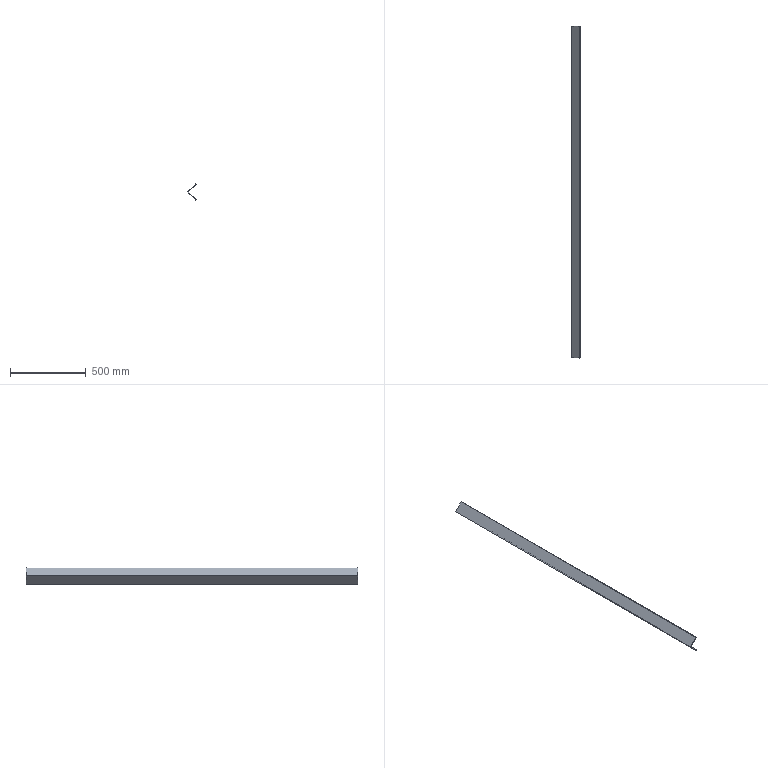Component | NX | CANTONEIRA | 1 solid | 12 faces | box 56.59 x 2190 x 106.11 mm | volume 1606510 mm3 | plane 8 | cylinder 4 | commonest cylinder face diameters 4 x4
STEP:
#1=CARTESIAN_POINT('',(0.,0.,0.));
#2=DIRECTION('',(0.,0.,1.));
#3=DIRECTION('',(1.,0.,0.));
#4=AXIS2_PLACEMENT_3D('',#1,#2,#3);
#5=CARTESIAN_POINT('',(-19.121,755.233,574.48));
#6=VERTEX_POINT('',#5);
#7=CARTESIAN_POINT('',(-71.589,755.233,626.947));
#8=VERTEX_POINT('',#7);
#9=CARTESIAN_POINT('',(-17.707,755.233,573.065));
#10=DIRECTION('',(-0.7071,0.,0.7071));
#11=VECTOR('',#10,1.);
#12=LINE('',#9,#11);
#13=CARTESIAN_POINT('',(-17.707,755.233,573.065));
#14=DIRECTION('',(0.7071,0.,0.7071));
#15=DIRECTION('',(-0.7071,0.,0.7071));
#16=AXIS2_PLACEMENT_3D('',#13,#14,#15);
#17=PLANE('',#16);
#18=CARTESIAN_POINT('',(0.,0.));
#19=DIRECTION('',(1.,0.));
#20=VECTOR('',#19,1.);
#21=LINE('',#18,#20);
#22=(GEOMETRIC_REPRESENTATION_CONTEXT(2)PARAMETRIC_REPRESENTATION_CONTEXT()REPRESENTATION_CONTEXT('',''));
#23=DEFINITIONAL_REPRESENTATION('',(#21),#22);
#24=PCURVE('',#17,#23);
#25=CARTESIAN_POINT('',(-71.589,755.233,626.947));
#26=DIRECTION('',(0.,1.,0.));
#27=DIRECTION('',(-0.7071,0.,0.7071));
#28=AXIS2_PLACEMENT_3D('',#25,#26,#27);
#29=PLANE('',#28);
#30=CARTESIAN_POINT('',(-76.2,0.));
#31=DIRECTION('',(1.,0.));
#32=VECTOR('',#31,1.);
#33=LINE('',#30,#32);
#34=(GEOMETRIC_REPRESENTATION_CONTEXT(2)PARAMETRIC_REPRESENTATION_CONTEXT()REPRESENTATION_CONTEXT('',''));
#35=DEFINITIONAL_REPRESENTATION('',(#33),#34);
#36=PCURVE('',#29,#35);
#37=SURFACE_CURVE('',#12,(#24,#36),.PCURVE_S1.);
#38=EDGE_CURVE('',#6,#8,#37,.T.);
#39=ORIENTED_EDGE('',*,*,#38,.F.);
#40=CARTESIAN_POINT('',(-19.121,-1434.767,574.48));
#41=VERTEX_POINT('',#40);
#42=CARTESIAN_POINT('',(-19.121,755.233,574.48));
#43=DIRECTION('',(0.,-1.,0.));
#44=VECTOR('',#43,1.);
#45=LINE('',#42,#44);
#46=CARTESIAN_POINT('',(2.,0.));
#47=DIRECTION('',(0.,1.));
#48=VECTOR('',#47,1.);
#49=LINE('',#46,#48);
#50=(GEOMETRIC_REPRESENTATION_CONTEXT(2)PARAMETRIC_REPRESENTATION_CONTEXT()REPRESENTATION_CONTEXT('',''));
#51=DEFINITIONAL_REPRESENTATION('',(#49),#50);
#52=PCURVE('',#17,#51);
#53=CARTESIAN_POINT('',(-17.707,755.233,575.894));
#54=DIRECTION('',(0.,-1.,0.));
#55=DIRECTION('',(0.7071,0.,-0.7071));
#56=AXIS2_PLACEMENT_3D('',#53,#54,#55);
#57=CYLINDRICAL_SURFACE('',#56,2.);
#58=CARTESIAN_POINT('',(4.712,0.));
#59=DIRECTION('',(0.,1.));
#60=VECTOR('',#59,1.);
#61=LINE('',#58,#60);
#62=(GEOMETRIC_REPRESENTATION_CONTEXT(2)PARAMETRIC_REPRESENTATION_CONTEXT()REPRESENTATION_CONTEXT('',''));
#63=DEFINITIONAL_REPRESENTATION('',(#61),#62);
#64=PCURVE('',#57,#63);
#65=SURFACE_CURVE('',#45,(#52,#64),.PCURVE_S1.);
#66=EDGE_CURVE('',#6,#41,#65,.T.);
#67=ORIENTED_EDGE('',*,*,#66,.T.);
#68=CARTESIAN_POINT('',(-71.589,-1434.767,626.947));
#69=VERTEX_POINT('',#68);
#70=CARTESIAN_POINT('',(-17.707,-1434.767,573.065));
#71=DIRECTION('',(-0.7071,0.,0.7071));
#72=VECTOR('',#71,1.);
#73=LINE('',#70,#72);
#74=CARTESIAN_POINT('',(0.,2190.));
#75=DIRECTION('',(1.,0.));
#76=VECTOR('',#75,1.);
#77=LINE('',#74,#76);
#78=(GEOMETRIC_REPRESENTATION_CONTEXT(2)PARAMETRIC_REPRESENTATION_CONTEXT()REPRESENTATION_CONTEXT('',''));
#79=DEFINITIONAL_REPRESENTATION('',(#77),#78);
#80=PCURVE('',#17,#79);
#81=CARTESIAN_POINT('',(-71.589,-1434.767,626.947));
#82=DIRECTION('',(0.,1.,0.));
#83=DIRECTION('',(-0.7071,0.,0.7071));
#84=AXIS2_PLACEMENT_3D('',#81,#82,#83);
#85=PLANE('',#84);
#86=CARTESIAN_POINT('',(-76.2,0.));
#87=DIRECTION('',(1.,0.));
#88=VECTOR('',#87,1.);
#89=LINE('',#86,#88);
#90=(GEOMETRIC_REPRESENTATION_CONTEXT(2)PARAMETRIC_REPRESENTATION_CONTEXT()REPRESENTATION_CONTEXT('',''));
#91=DEFINITIONAL_REPRESENTATION('',(#89),#90);
#92=PCURVE('',#85,#91);
#93=SURFACE_CURVE('',#73,(#80,#92),.PCURVE_S1.);
#94=EDGE_CURVE('',#41,#69,#93,.T.);
#95=ORIENTED_EDGE('',*,*,#94,.T.);
#96=CARTESIAN_POINT('',(-71.589,755.233,626.947));
#97=DIRECTION('',(0.,-1.,0.));
#98=VECTOR('',#97,1.);
#99=LINE('',#96,#98);
#100=CARTESIAN_POINT('',(76.2,0.));
#101=DIRECTION('',(0.,1.));
#102=VECTOR('',#101,1.);
#103=LINE('',#100,#102);
#104=(GEOMETRIC_REPRESENTATION_CONTEXT(2)PARAMETRIC_REPRESENTATION_CONTEXT()REPRESENTATION_CONTEXT('',''));
#105=DEFINITIONAL_REPRESENTATION('',(#103),#104);
#106=PCURVE('',#17,#105);
#107=CARTESIAN_POINT('',(-71.589,755.233,626.947));
#108=DIRECTION('',(0.7071,0.,-0.7071));
#109=DIRECTION('',(0.7071,0.,0.7071));
#110=AXIS2_PLACEMENT_3D('',#107,#108,#109);
#111=PLANE('',#110);
#112=CARTESIAN_POINT('',(0.,0.));
#113=DIRECTION('',(0.,1.));
#114=VECTOR('',#113,1.);
#115=LINE('',#112,#114);
#116=(GEOMETRIC_REPRESENTATION_CONTEXT(2)PARAMETRIC_REPRESENTATION_CONTEXT()REPRESENTATION_CONTEXT('',''));
#117=DEFINITIONAL_REPRESENTATION('',(#115),#116);
#118=PCURVE('',#111,#117);
#119=SURFACE_CURVE('',#99,(#106,#118),.PCURVE_S1.);
#120=EDGE_CURVE('',#8,#69,#119,.T.);
#121=ORIENTED_EDGE('',*,*,#120,.F.);
#122=EDGE_LOOP('',(#39,#67,#95,#121));
#123=FACE_BOUND('',#122,.T.);
#124=ADVANCED_FACE('',(#123),#17,.F.);
#125=CARTESIAN_POINT('',(-19.121,-1434.767,679.414));
#126=VERTEX_POINT('',#125);
#127=CARTESIAN_POINT('',(-71.589,-1434.767,626.947));
#128=DIRECTION('',(0.7071,0.,0.7071));
#129=VECTOR('',#128,1.);
#130=LINE('',#127,#129);
#131=CARTESIAN_POINT('',(0.,2190.));
#132=DIRECTION('',(1.,0.));
#133=VECTOR('',#132,1.);
#134=LINE('',#131,#133);
#135=(GEOMETRIC_REPRESENTATION_CONTEXT(2)PARAMETRIC_REPRESENTATION_CONTEXT()REPRESENTATION_CONTEXT('',''));
#136=DEFINITIONAL_REPRESENTATION('',(#134),#135);
#137=PCURVE('',#111,#136);
#138=CARTESIAN_POINT('',(0.,0.));
#139=DIRECTION('',(0.,1.));
#140=VECTOR('',#139,1.);
#141=LINE('',#138,#140);
#142=(GEOMETRIC_REPRESENTATION_CONTEXT(2)PARAMETRIC_REPRESENTATION_CONTEXT()REPRESENTATION_CONTEXT('',''));
#143=DEFINITIONAL_REPRESENTATION('',(#141),#142);
#144=PCURVE('',#85,#143);
#145=SURFACE_CURVE('',#130,(#137,#144),.PCURVE_S1.);
#146=EDGE_CURVE('',#69,#126,#145,.T.);
#147=ORIENTED_EDGE('',*,*,#146,.T.);
#148=CARTESIAN_POINT('',(-19.121,755.233,679.414));
#149=VERTEX_POINT('',#148);
#150=CARTESIAN_POINT('',(-19.121,755.233,679.414));
#151=DIRECTION('',(0.,1.,0.));
#152=VECTOR('',#151,1.);
#153=LINE('',#150,#152);
#154=CARTESIAN_POINT('',(74.2,0.));
#155=DIRECTION('',(0.,-1.));
#156=VECTOR('',#155,1.);
#157=LINE('',#154,#156);
#158=(GEOMETRIC_REPRESENTATION_CONTEXT(2)PARAMETRIC_REPRESENTATION_CONTEXT()REPRESENTATION_CONTEXT('',''));
#159=DEFINITIONAL_REPRESENTATION('',(#157),#158);
#160=PCURVE('',#111,#159);
#161=CARTESIAN_POINT('',(-17.707,755.233,678.));
#162=DIRECTION('',(0.,-1.,0.));
#163=DIRECTION('',(0.7071,0.,-0.7071));
#164=AXIS2_PLACEMENT_3D('',#161,#162,#163);
#165=CYLINDRICAL_SURFACE('',#164,2.);
#166=CARTESIAN_POINT('',(3.142,0.));
#167=DIRECTION('',(0.,-1.));
#168=VECTOR('',#167,1.);
#169=LINE('',#166,#168);
#170=(GEOMETRIC_REPRESENTATION_CONTEXT(2)PARAMETRIC_REPRESENTATION_CONTEXT()REPRESENTATION_CONTEXT('',''));
#171=DEFINITIONAL_REPRESENTATION('',(#169),#170);
#172=PCURVE('',#165,#171);
#173=SURFACE_CURVE('',#153,(#160,#172),.PCURVE_S1.);
#174=EDGE_CURVE('',#126,#149,#173,.T.);
#175=ORIENTED_EDGE('',*,*,#174,.T.);
#176=CARTESIAN_POINT('',(-71.589,755.233,626.947));
#177=DIRECTION('',(0.7071,0.,0.7071));
#178=VECTOR('',#177,1.);
#179=LINE('',#176,#178);
#180=CARTESIAN_POINT('',(0.,0.));
#181=DIRECTION('',(1.,0.));
#182=VECTOR('',#181,1.);
#183=LINE('',#180,#182);
#184=(GEOMETRIC_REPRESENTATION_CONTEXT(2)PARAMETRIC_REPRESENTATION_CONTEXT()REPRESENTATION_CONTEXT('',''));
#185=DEFINITIONAL_REPRESENTATION('',(#183),#184);
#186=PCURVE('',#111,#185);
#187=CARTESIAN_POINT('',(0.,0.));
#188=DIRECTION('',(0.,1.));
#189=VECTOR('',#188,1.);
#190=LINE('',#187,#189);
#191=(GEOMETRIC_REPRESENTATION_CONTEXT(2)PARAMETRIC_REPRESENTATION_CONTEXT()REPRESENTATION_CONTEXT('',''));
#192=DEFINITIONAL_REPRESENTATION('',(#190),#191);
#193=PCURVE('',#29,#192);
#194=SURFACE_CURVE('',#179,(#186,#193),.PCURVE_S1.);
#195=EDGE_CURVE('',#8,#149,#194,.T.);
#196=ORIENTED_EDGE('',*,*,#195,.F.);
#197=ORIENTED_EDGE('',*,*,#120,.T.);
#198=EDGE_LOOP('',(#147,#175,#196,#197));
#199=FACE_BOUND('',#198,.T.);
#200=ADVANCED_FACE('',(#199),#111,.F.);
#201=CARTESIAN_POINT('',(-16.293,755.233,679.414));
#202=VERTEX_POINT('',#201);
#203=CARTESIAN_POINT('',(-15.586,755.233,678.707));
#204=VERTEX_POINT('',#203);
#205=CARTESIAN_POINT('',(-17.707,755.233,680.828));
#206=DIRECTION('',(0.7071,0.,-0.7071));
#207=VECTOR('',#206,1.);
#208=LINE('',#205,#207);
#209=CARTESIAN_POINT('',(-17.707,755.233,680.828));
#210=DIRECTION('',(-0.7071,0.,-0.7071));
#211=DIRECTION('',(0.7071,0.,-0.7071));
#212=AXIS2_PLACEMENT_3D('',#209,#210,#211);
#213=PLANE('',#212);
#214=CARTESIAN_POINT('',(0.,0.));
#215=DIRECTION('',(1.,0.));
#216=VECTOR('',#215,1.);
#217=LINE('',#214,#216);
#218=(GEOMETRIC_REPRESENTATION_CONTEXT(2)PARAMETRIC_REPRESENTATION_CONTEXT()REPRESENTATION_CONTEXT('',''));
#219=DEFINITIONAL_REPRESENTATION('',(#217),#218);
#220=PCURVE('',#213,#219);
#221=CARTESIAN_POINT('',(-0.,76.2));
#222=DIRECTION('',(-1.,0.));
#223=VECTOR('',#222,1.);
#224=LINE('',#221,#223);
#225=(GEOMETRIC_REPRESENTATION_CONTEXT(2)PARAMETRIC_REPRESENTATION_CONTEXT()REPRESENTATION_CONTEXT('',''));
#226=DEFINITIONAL_REPRESENTATION('',(#224),#225);
#227=PCURVE('',#29,#226);
#228=SURFACE_CURVE('',#208,(#220,#227),.PCURVE_S1.);
#229=EDGE_CURVE('',#202,#204,#228,.T.);
#230=ORIENTED_EDGE('',*,*,#229,.F.);
#231=CARTESIAN_POINT('',(-16.293,-1434.767,679.414));
#232=VERTEX_POINT('',#231);
#233=CARTESIAN_POINT('',(-16.293,755.233,679.414));
#234=DIRECTION('',(0.,-1.,0.));
#235=VECTOR('',#234,1.);
#236=LINE('',#233,#235);
#237=CARTESIAN_POINT('',(2.,0.));
#238=DIRECTION('',(0.,1.));
#239=VECTOR('',#238,1.);
#240=LINE('',#237,#239);
#241=(GEOMETRIC_REPRESENTATION_CONTEXT(2)PARAMETRIC_REPRESENTATION_CONTEXT()REPRESENTATION_CONTEXT('',''));
#242=DEFINITIONAL_REPRESENTATION('',(#240),#241);
#243=PCURVE('',#213,#242);
#244=CARTESIAN_POINT('',(1.571,0.));
#245=DIRECTION('',(0.,1.));
#246=VECTOR('',#245,1.);
#247=LINE('',#244,#246);
#248=(GEOMETRIC_REPRESENTATION_CONTEXT(2)PARAMETRIC_REPRESENTATION_CONTEXT()REPRESENTATION_CONTEXT('',''));
#249=DEFINITIONAL_REPRESENTATION('',(#247),#248);
#250=PCURVE('',#165,#249);
#251=SURFACE_CURVE('',#236,(#243,#250),.PCURVE_S1.);
#252=EDGE_CURVE('',#202,#232,#251,.T.);
#253=ORIENTED_EDGE('',*,*,#252,.T.);
#254=CARTESIAN_POINT('',(-15.586,-1434.767,678.707));
#255=VERTEX_POINT('',#254);
#256=CARTESIAN_POINT('',(-17.707,-1434.767,680.828));
#257=DIRECTION('',(0.7071,0.,-0.7071));
#258=VECTOR('',#257,1.);
#259=LINE('',#256,#258);
#260=CARTESIAN_POINT('',(0.,2190.));
#261=DIRECTION('',(1.,0.));
#262=VECTOR('',#261,1.);
#263=LINE('',#260,#262);
#264=(GEOMETRIC_REPRESENTATION_CONTEXT(2)PARAMETRIC_REPRESENTATION_CONTEXT()REPRESENTATION_CONTEXT('',''));
#265=DEFINITIONAL_REPRESENTATION('',(#263),#264);
#266=PCURVE('',#213,#265);
#267=CARTESIAN_POINT('',(-0.,76.2));
#268=DIRECTION('',(-1.,0.));
#269=VECTOR('',#268,1.);
#270=LINE('',#267,#269);
#271=(GEOMETRIC_REPRESENTATION_CONTEXT(2)PARAMETRIC_REPRESENTATION_CONTEXT()REPRESENTATION_CONTEXT('',''));
#272=DEFINITIONAL_REPRESENTATION('',(#270),#271);
#273=PCURVE('',#85,#272);
#274=SURFACE_CURVE('',#259,(#266,#273),.PCURVE_S1.);
#275=EDGE_CURVE('',#232,#255,#274,.T.);
#276=ORIENTED_EDGE('',*,*,#275,.T.);
#277=CARTESIAN_POINT('',(-15.586,755.233,678.707));
#278=DIRECTION('',(0.,1.,0.));
#279=VECTOR('',#278,1.);
#280=LINE('',#277,#279);
#281=CARTESIAN_POINT('',(3.,0.));
#282=DIRECTION('',(0.,-1.));
#283=VECTOR('',#282,1.);
#284=LINE('',#281,#283);
#285=(GEOMETRIC_REPRESENTATION_CONTEXT(2)PARAMETRIC_REPRESENTATION_CONTEXT()REPRESENTATION_CONTEXT('',''));
#286=DEFINITIONAL_REPRESENTATION('',(#284),#285);
#287=PCURVE('',#213,#286);
#288=CARTESIAN_POINT('',(-17.,755.233,677.293));
#289=DIRECTION('',(0.,-1.,0.));
#290=DIRECTION('',(0.7071,0.,-0.7071));
#291=AXIS2_PLACEMENT_3D('',#288,#289,#290);
#292=CYLINDRICAL_SURFACE('',#291,2.);
#293=CARTESIAN_POINT('',(1.571,0.));
#294=DIRECTION('',(0.,-1.));
#295=VECTOR('',#294,1.);
#296=LINE('',#293,#295);
#297=(GEOMETRIC_REPRESENTATION_CONTEXT(2)PARAMETRIC_REPRESENTATION_CONTEXT()REPRESENTATION_CONTEXT('',''));
#298=DEFINITIONAL_REPRESENTATION('',(#296),#297);
#299=PCURVE('',#292,#298);
#300=SURFACE_CURVE('',#280,(#287,#299),.PCURVE_S1.);
#301=EDGE_CURVE('',#255,#204,#300,.T.);
#302=ORIENTED_EDGE('',*,*,#301,.T.);
#303=EDGE_LOOP('',(#230,#253,#276,#302));
#304=FACE_BOUND('',#303,.T.);
#305=ADVANCED_FACE('',(#304),#213,.F.);
#306=CARTESIAN_POINT('',(-15.586,755.233,675.879));
#307=VERTEX_POINT('',#306);
#308=CARTESIAN_POINT('',(-64.518,755.233,626.947));
#309=VERTEX_POINT('',#308);
#310=CARTESIAN_POINT('',(-14.172,755.233,677.293));
#311=DIRECTION('',(-0.7071,0.,-0.7071));
#312=VECTOR('',#311,1.);
#313=LINE('',#310,#312);
#314=CARTESIAN_POINT('',(-14.172,755.233,677.293));
#315=DIRECTION('',(-0.7071,0.,0.7071));
#316=DIRECTION('',(-0.7071,0.,-0.7071));
#317=AXIS2_PLACEMENT_3D('',#314,#315,#316);
#318=PLANE('',#317);
#319=CARTESIAN_POINT('',(0.,0.));
#320=DIRECTION('',(1.,0.));
#321=VECTOR('',#320,1.);
#322=LINE('',#319,#321);
#323=(GEOMETRIC_REPRESENTATION_CONTEXT(2)PARAMETRIC_REPRESENTATION_CONTEXT()REPRESENTATION_CONTEXT('',''));
#324=DEFINITIONAL_REPRESENTATION('',(#322),#323);
#325=PCURVE('',#318,#324);
#326=CARTESIAN_POINT('',(-5.,76.2));
#327=DIRECTION('',(0.,-1.));
#328=VECTOR('',#327,1.);
#329=LINE('',#326,#328);
#330=(GEOMETRIC_REPRESENTATION_CONTEXT(2)PARAMETRIC_REPRESENTATION_CONTEXT()REPRESENTATION_CONTEXT('',''));
#331=DEFINITIONAL_REPRESENTATION('',(#329),#330);
#332=PCURVE('',#29,#331);
#333=SURFACE_CURVE('',#313,(#325,#332),.PCURVE_S1.);
#334=EDGE_CURVE('',#307,#309,#333,.T.);
#335=ORIENTED_EDGE('',*,*,#334,.F.);
#336=CARTESIAN_POINT('',(-15.586,-1434.767,675.879));
#337=VERTEX_POINT('',#336);
#338=CARTESIAN_POINT('',(-15.586,755.233,675.879));
#339=DIRECTION('',(0.,-1.,0.));
#340=VECTOR('',#339,1.);
#341=LINE('',#338,#340);
#342=CARTESIAN_POINT('',(2.,0.));
#343=DIRECTION('',(0.,1.));
#344=VECTOR('',#343,1.);
#345=LINE('',#342,#344);
#346=(GEOMETRIC_REPRESENTATION_CONTEXT(2)PARAMETRIC_REPRESENTATION_CONTEXT()REPRESENTATION_CONTEXT('',''));
#347=DEFINITIONAL_REPRESENTATION('',(#345),#346);
#348=PCURVE('',#318,#347);
#349=CARTESIAN_POINT('',(0.,0.));
#350=DIRECTION('',(0.,1.));
#351=VECTOR('',#350,1.);
#352=LINE('',#349,#351);
#353=(GEOMETRIC_REPRESENTATION_CONTEXT(2)PARAMETRIC_REPRESENTATION_CONTEXT()REPRESENTATION_CONTEXT('',''));
#354=DEFINITIONAL_REPRESENTATION('',(#352),#353);
#355=PCURVE('',#292,#354);
#356=SURFACE_CURVE('',#341,(#348,#355),.PCURVE_S1.);
#357=EDGE_CURVE('',#307,#337,#356,.T.);
#358=ORIENTED_EDGE('',*,*,#357,.T.);
#359=CARTESIAN_POINT('',(-64.518,-1434.767,626.947));
#360=VERTEX_POINT('',#359);
#361=CARTESIAN_POINT('',(-14.172,-1434.767,677.293));
#362=DIRECTION('',(-0.7071,0.,-0.7071));
#363=VECTOR('',#362,1.);
#364=LINE('',#361,#363);
#365=CARTESIAN_POINT('',(0.,2190.));
#366=DIRECTION('',(1.,0.));
#367=VECTOR('',#366,1.);
#368=LINE('',#365,#367);
#369=(GEOMETRIC_REPRESENTATION_CONTEXT(2)PARAMETRIC_REPRESENTATION_CONTEXT()REPRESENTATION_CONTEXT('',''));
#370=DEFINITIONAL_REPRESENTATION('',(#368),#369);
#371=PCURVE('',#318,#370);
#372=CARTESIAN_POINT('',(-5.,76.2));
#373=DIRECTION('',(0.,-1.));
#374=VECTOR('',#373,1.);
#375=LINE('',#372,#374);
#376=(GEOMETRIC_REPRESENTATION_CONTEXT(2)PARAMETRIC_REPRESENTATION_CONTEXT()REPRESENTATION_CONTEXT('',''));
#377=DEFINITIONAL_REPRESENTATION('',(#375),#376);
#378=PCURVE('',#85,#377);
#379=SURFACE_CURVE('',#364,(#371,#378),.PCURVE_S1.);
#380=EDGE_CURVE('',#337,#360,#379,.T.);
#381=ORIENTED_EDGE('',*,*,#380,.T.);
#382=CARTESIAN_POINT('',(-64.518,755.233,626.947));
#383=DIRECTION('',(0.,-1.,0.));
#384=VECTOR('',#383,1.);
#385=LINE('',#382,#384);
#386=CARTESIAN_POINT('',(71.2,0.));
#387=DIRECTION('',(0.,1.));
#388=VECTOR('',#387,1.);
#389=LINE('',#386,#388);
#390=(GEOMETRIC_REPRESENTATION_CONTEXT(2)PARAMETRIC_REPRESENTATION_CONTEXT()REPRESENTATION_CONTEXT('',''));
#391=DEFINITIONAL_REPRESENTATION('',(#389),#390);
#392=PCURVE('',#318,#391);
#393=CARTESIAN_POINT('',(-64.518,755.233,626.947));
#394=DIRECTION('',(-0.7071,0.,-0.7071));
#395=DIRECTION('',(0.7071,0.,-0.7071));
#396=AXIS2_PLACEMENT_3D('',#393,#394,#395);
#397=PLANE('',#396);
#398=CARTESIAN_POINT('',(0.,0.));
#399=DIRECTION('',(0.,1.));
#400=VECTOR('',#399,1.);
#401=LINE('',#398,#400);
#402=(GEOMETRIC_REPRESENTATION_CONTEXT(2)PARAMETRIC_REPRESENTATION_CONTEXT()REPRESENTATION_CONTEXT('',''));
#403=DEFINITIONAL_REPRESENTATION('',(#401),#402);
#404=PCURVE('',#397,#403);
#405=SURFACE_CURVE('',#385,(#392,#404),.PCURVE_S1.);
#406=EDGE_CURVE('',#309,#360,#405,.T.);
#407=ORIENTED_EDGE('',*,*,#406,.F.);
#408=EDGE_LOOP('',(#335,#358,#381,#407));
#409=FACE_BOUND('',#408,.T.);
#410=ADVANCED_FACE('',(#409),#318,.F.);
#411=CARTESIAN_POINT('',(-15.586,-1434.767,578.015));
#412=VERTEX_POINT('',#411);
#413=CARTESIAN_POINT('',(-64.518,-1434.767,626.947));
#414=DIRECTION('',(0.7071,0.,-0.7071));
#415=VECTOR('',#414,1.);
#416=LINE('',#413,#415);
#417=CARTESIAN_POINT('',(0.,2190.));
#418=DIRECTION('',(1.,0.));
#419=VECTOR('',#418,1.);
#420=LINE('',#417,#419);
#421=(GEOMETRIC_REPRESENTATION_CONTEXT(2)PARAMETRIC_REPRESENTATION_CONTEXT()REPRESENTATION_CONTEXT('',''));
#422=DEFINITIONAL_REPRESENTATION('',(#420),#421);
#423=PCURVE('',#397,#422);
#424=CARTESIAN_POINT('',(-5.,5.));
#425=DIRECTION('',(-1.,0.));
#426=VECTOR('',#425,1.);
#427=LINE('',#424,#426);
#428=(GEOMETRIC_REPRESENTATION_CONTEXT(2)PARAMETRIC_REPRESENTATION_CONTEXT()REPRESENTATION_CONTEXT('',''));
#429=DEFINITIONAL_REPRESENTATION('',(#427),#428);
#430=PCURVE('',#85,#429);
#431=SURFACE_CURVE('',#416,(#423,#430),.PCURVE_S1.);
#432=EDGE_CURVE('',#360,#412,#431,.T.);
#433=ORIENTED_EDGE('',*,*,#432,.T.);
#434=CARTESIAN_POINT('',(-15.586,755.233,578.015));
#435=VERTEX_POINT('',#434);
#436=CARTESIAN_POINT('',(-15.586,755.233,578.015));
#437=DIRECTION('',(0.,1.,0.));
#438=VECTOR('',#437,1.);
#439=LINE('',#436,#438);
#440=CARTESIAN_POINT('',(69.2,0.));
#441=DIRECTION('',(0.,-1.));
#442=VECTOR('',#441,1.);
#443=LINE('',#440,#442);
#444=(GEOMETRIC_REPRESENTATION_CONTEXT(2)PARAMETRIC_REPRESENTATION_CONTEXT()REPRESENTATION_CONTEXT('',''));
#445=DEFINITIONAL_REPRESENTATION('',(#443),#444);
#446=PCURVE('',#397,#445);
#447=CARTESIAN_POINT('',(-17.,755.233,576.601));
#448=DIRECTION('',(0.,-1.,0.));
#449=DIRECTION('',(0.7071,0.,-0.7071));
#450=AXIS2_PLACEMENT_3D('',#447,#448,#449);
#451=CYLINDRICAL_SURFACE('',#450,2.);
#452=CARTESIAN_POINT('',(1.571,0.));
#453=DIRECTION('',(0.,-1.));
#454=VECTOR('',#453,1.);
#455=LINE('',#452,#454);
#456=(GEOMETRIC_REPRESENTATION_CONTEXT(2)PARAMETRIC_REPRESENTATION_CONTEXT()REPRESENTATION_CONTEXT('',''));
#457=DEFINITIONAL_REPRESENTATION('',(#455),#456);
#458=PCURVE('',#451,#457);
#459=SURFACE_CURVE('',#439,(#446,#458),.PCURVE_S1.);
#460=EDGE_CURVE('',#412,#435,#459,.T.);
#461=ORIENTED_EDGE('',*,*,#460,.T.);
#462=CARTESIAN_POINT('',(-64.518,755.233,626.947));
#463=DIRECTION('',(0.7071,0.,-0.7071));
#464=VECTOR('',#463,1.);
#465=LINE('',#462,#464);
#466=CARTESIAN_POINT('',(0.,0.));
#467=DIRECTION('',(1.,0.));
#468=VECTOR('',#467,1.);
#469=LINE('',#466,#468);
#470=(GEOMETRIC_REPRESENTATION_CONTEXT(2)PARAMETRIC_REPRESENTATION_CONTEXT()REPRESENTATION_CONTEXT('',''));
#471=DEFINITIONAL_REPRESENTATION('',(#469),#470);
#472=PCURVE('',#397,#471);
#473=CARTESIAN_POINT('',(-5.,5.));
#474=DIRECTION('',(-1.,0.));
#475=VECTOR('',#474,1.);
#476=LINE('',#473,#475);
#477=(GEOMETRIC_REPRESENTATION_CONTEXT(2)PARAMETRIC_REPRESENTATION_CONTEXT()REPRESENTATION_CONTEXT('',''));
#478=DEFINITIONAL_REPRESENTATION('',(#476),#477);
#479=PCURVE('',#29,#478);
#480=SURFACE_CURVE('',#465,(#472,#479),.PCURVE_S1.);
#481=EDGE_CURVE('',#309,#435,#480,.T.);
#482=ORIENTED_EDGE('',*,*,#481,.F.);
#483=ORIENTED_EDGE('',*,*,#406,.T.);
#484=EDGE_LOOP('',(#433,#461,#482,#483));
#485=FACE_BOUND('',#484,.T.);
#486=ADVANCED_FACE('',(#485),#397,.F.);
#487=CARTESIAN_POINT('',(-15.586,755.233,575.187));
#488=VERTEX_POINT('',#487);
#489=CARTESIAN_POINT('',(-16.293,755.233,574.48));
#490=VERTEX_POINT('',#489);
#491=CARTESIAN_POINT('',(-14.172,755.233,576.601));
#492=DIRECTION('',(-0.7071,0.,-0.7071));
#493=VECTOR('',#492,1.);
#494=LINE('',#491,#493);
#495=CARTESIAN_POINT('',(-14.172,755.233,576.601));
#496=DIRECTION('',(-0.7071,0.,0.7071));
#497=DIRECTION('',(-0.7071,0.,-0.7071));
#498=AXIS2_PLACEMENT_3D('',#495,#496,#497);
#499=PLANE('',#498);
#500=CARTESIAN_POINT('',(0.,0.));
#501=DIRECTION('',(1.,0.));
#502=VECTOR('',#501,1.);
#503=LINE('',#500,#502);
#504=(GEOMETRIC_REPRESENTATION_CONTEXT(2)PARAMETRIC_REPRESENTATION_CONTEXT()REPRESENTATION_CONTEXT('',''));
#505=DEFINITIONAL_REPRESENTATION('',(#503),#504);
#506=PCURVE('',#499,#505);
#507=CARTESIAN_POINT('',(-76.2,5.));
#508=DIRECTION('',(0.,-1.));
#509=VECTOR('',#508,1.);
#510=LINE('',#507,#509);
#511=(GEOMETRIC_REPRESENTATION_CONTEXT(2)PARAMETRIC_REPRESENTATION_CONTEXT()REPRESENTATION_CONTEXT('',''));
#512=DEFINITIONAL_REPRESENTATION('',(#510),#511);
#513=PCURVE('',#29,#512);
#514=SURFACE_CURVE('',#494,(#506,#513),.PCURVE_S1.);
#515=EDGE_CURVE('',#488,#490,#514,.T.);
#516=ORIENTED_EDGE('',*,*,#515,.F.);
#517=CARTESIAN_POINT('',(-15.586,-1434.767,575.187));
#518=VERTEX_POINT('',#517);
#519=CARTESIAN_POINT('',(-15.586,755.233,575.187));
#520=DIRECTION('',(0.,-1.,0.));
#521=VECTOR('',#520,1.);
#522=LINE('',#519,#521);
#523=CARTESIAN_POINT('',(2.,0.));
#524=DIRECTION('',(0.,1.));
#525=VECTOR('',#524,1.);
#526=LINE('',#523,#525);
#527=(GEOMETRIC_REPRESENTATION_CONTEXT(2)PARAMETRIC_REPRESENTATION_CONTEXT()REPRESENTATION_CONTEXT('',''));
#528=DEFINITIONAL_REPRESENTATION('',(#526),#527);
#529=PCURVE('',#499,#528);
#530=CARTESIAN_POINT('',(0.,0.));
#531=DIRECTION('',(0.,1.));
#532=VECTOR('',#531,1.);
#533=LINE('',#530,#532);
#534=(GEOMETRIC_REPRESENTATION_CONTEXT(2)PARAMETRIC_REPRESENTATION_CONTEXT()REPRESENTATION_CONTEXT('',''));
#535=DEFINITIONAL_REPRESENTATION('',(#533),#534);
#536=PCURVE('',#451,#535);
#537=SURFACE_CURVE('',#522,(#529,#536),.PCURVE_S1.);
#538=EDGE_CURVE('',#488,#518,#537,.T.);
#539=ORIENTED_EDGE('',*,*,#538,.T.);
#540=CARTESIAN_POINT('',(-16.293,-1434.767,574.48));
#541=VERTEX_POINT('',#540);
#542=CARTESIAN_POINT('',(-14.172,-1434.767,576.601));
#543=DIRECTION('',(-0.7071,0.,-0.7071));
#544=VECTOR('',#543,1.);
#545=LINE('',#542,#544);
#546=CARTESIAN_POINT('',(0.,2190.));
#547=DIRECTION('',(1.,0.));
#548=VECTOR('',#547,1.);
#549=LINE('',#546,#548);
#550=(GEOMETRIC_REPRESENTATION_CONTEXT(2)PARAMETRIC_REPRESENTATION_CONTEXT()REPRESENTATION_CONTEXT('',''));
#551=DEFINITIONAL_REPRESENTATION('',(#549),#550);
#552=PCURVE('',#499,#551);
#553=CARTESIAN_POINT('',(-76.2,5.));
#554=DIRECTION('',(0.,-1.));
#555=VECTOR('',#554,1.);
#556=LINE('',#553,#555);
#557=(GEOMETRIC_REPRESENTATION_CONTEXT(2)PARAMETRIC_REPRESENTATION_CONTEXT()REPRESENTATION_CONTEXT('',''));
#558=DEFINITIONAL_REPRESENTATION('',(#556),#557);
#559=PCURVE('',#85,#558);
#560=SURFACE_CURVE('',#545,(#552,#559),.PCURVE_S1.);
#561=EDGE_CURVE('',#518,#541,#560,.T.);
#562=ORIENTED_EDGE('',*,*,#561,.T.);
#563=CARTESIAN_POINT('',(-16.293,755.233,574.48));
#564=DIRECTION('',(0.,1.,0.));
#565=VECTOR('',#564,1.);
#566=LINE('',#563,#565);
#567=CARTESIAN_POINT('',(3.,0.));
#568=DIRECTION('',(0.,-1.));
#569=VECTOR('',#568,1.);
#570=LINE('',#567,#569);
#571=(GEOMETRIC_REPRESENTATION_CONTEXT(2)PARAMETRIC_REPRESENTATION_CONTEXT()REPRESENTATION_CONTEXT('',''));
#572=DEFINITIONAL_REPRESENTATION('',(#570),#571);
#573=PCURVE('',#499,#572);
#574=CARTESIAN_POINT('',(6.283,0.));
#575=DIRECTION('',(0.,-1.));
#576=VECTOR('',#575,1.);
#577=LINE('',#574,#576);
#578=(GEOMETRIC_REPRESENTATION_CONTEXT(2)PARAMETRIC_REPRESENTATION_CONTEXT()REPRESENTATION_CONTEXT('',''));
#579=DEFINITIONAL_REPRESENTATION('',(#577),#578);
#580=PCURVE('',#57,#579);
#581=SURFACE_CURVE('',#566,(#573,#580),.PCURVE_S1.);
#582=EDGE_CURVE('',#541,#490,#581,.T.);
#583=ORIENTED_EDGE('',*,*,#582,.T.);
#584=EDGE_LOOP('',(#516,#539,#562,#583));
#585=FACE_BOUND('',#584,.T.);
#586=ADVANCED_FACE('',(#585),#499,.F.);
#587=ORIENTED_EDGE('',*,*,#195,.T.);
#588=CARTESIAN_POINT('',(-17.707,755.233,678.));
#589=DIRECTION('',(0.,1.,0.));
#590=DIRECTION('',(-0.7071,0.,0.7071));
#591=AXIS2_PLACEMENT_3D('',#588,#589,#590);
#592=CIRCLE('',#591,2.);
#593=CARTESIAN_POINT('',(-2.,74.2));
#594=DIRECTION('',(1.,0.));
#595=AXIS2_PLACEMENT_2D('',#593,#594);
#596=CIRCLE('',#595,2.);
#597=(GEOMETRIC_REPRESENTATION_CONTEXT(2)PARAMETRIC_REPRESENTATION_CONTEXT()REPRESENTATION_CONTEXT('',''));
#598=DEFINITIONAL_REPRESENTATION('',(#596),#597);
#599=PCURVE('',#29,#598);
#600=CARTESIAN_POINT('',(3.142,0.));
#601=DIRECTION('',(-1.,0.));
#602=VECTOR('',#601,1.);
#603=LINE('',#600,#602);
#604=(GEOMETRIC_REPRESENTATION_CONTEXT(2)PARAMETRIC_REPRESENTATION_CONTEXT()REPRESENTATION_CONTEXT('',''));
#605=DEFINITIONAL_REPRESENTATION('',(#603),#604);
#606=PCURVE('',#165,#605);
#607=SURFACE_CURVE('',#592,(#599,#606),.PCURVE_S1.);
#608=EDGE_CURVE('',#149,#202,#607,.T.);
#609=ORIENTED_EDGE('',*,*,#608,.T.);
#610=ORIENTED_EDGE('',*,*,#229,.T.);
#611=CARTESIAN_POINT('',(-17.,755.233,677.293));
#612=DIRECTION('',(0.,1.,0.));
#613=DIRECTION('',(-0.7071,0.,0.7071));
#614=AXIS2_PLACEMENT_3D('',#611,#612,#613);
#615=CIRCLE('',#614,2.);
#616=CARTESIAN_POINT('',(-3.,74.2));
#617=DIRECTION('',(1.,0.));
#618=AXIS2_PLACEMENT_2D('',#616,#617);
#619=CIRCLE('',#618,2.);
#620=(GEOMETRIC_REPRESENTATION_CONTEXT(2)PARAMETRIC_REPRESENTATION_CONTEXT()REPRESENTATION_CONTEXT('',''));
#621=DEFINITIONAL_REPRESENTATION('',(#619),#620);
#622=PCURVE('',#29,#621);
#623=CARTESIAN_POINT('',(3.142,0.));
#624=DIRECTION('',(-1.,0.));
#625=VECTOR('',#624,1.);
#626=LINE('',#623,#625);
#627=(GEOMETRIC_REPRESENTATION_CONTEXT(2)PARAMETRIC_REPRESENTATION_CONTEXT()REPRESENTATION_CONTEXT('',''));
#628=DEFINITIONAL_REPRESENTATION('',(#626),#627);
#629=PCURVE('',#292,#628);
#630=SURFACE_CURVE('',#615,(#622,#629),.PCURVE_S1.);
#631=EDGE_CURVE('',#204,#307,#630,.T.);
#632=ORIENTED_EDGE('',*,*,#631,.T.);
#633=ORIENTED_EDGE('',*,*,#334,.T.);
#634=ORIENTED_EDGE('',*,*,#481,.T.);
#635=CARTESIAN_POINT('',(-17.,755.233,576.601));
#636=DIRECTION('',(0.,1.,0.));
#637=DIRECTION('',(-0.7071,0.,0.7071));
#638=AXIS2_PLACEMENT_3D('',#635,#636,#637);
#639=CIRCLE('',#638,2.);
#640=CARTESIAN_POINT('',(-74.2,3.));
#641=DIRECTION('',(1.,0.));
#642=AXIS2_PLACEMENT_2D('',#640,#641);
#643=CIRCLE('',#642,2.);
#644=(GEOMETRIC_REPRESENTATION_CONTEXT(2)PARAMETRIC_REPRESENTATION_CONTEXT()REPRESENTATION_CONTEXT('',''));
#645=DEFINITIONAL_REPRESENTATION('',(#643),#644);
#646=PCURVE('',#29,#645);
#647=CARTESIAN_POINT('',(3.142,0.));
#648=DIRECTION('',(-1.,0.));
#649=VECTOR('',#648,1.);
#650=LINE('',#647,#649);
#651=(GEOMETRIC_REPRESENTATION_CONTEXT(2)PARAMETRIC_REPRESENTATION_CONTEXT()REPRESENTATION_CONTEXT('',''));
#652=DEFINITIONAL_REPRESENTATION('',(#650),#651);
#653=PCURVE('',#451,#652);
#654=SURFACE_CURVE('',#639,(#646,#653),.PCURVE_S1.);
#655=EDGE_CURVE('',#435,#488,#654,.T.);
#656=ORIENTED_EDGE('',*,*,#655,.T.);
#657=ORIENTED_EDGE('',*,*,#515,.T.);
#658=CARTESIAN_POINT('',(-17.707,755.233,575.894));
#659=DIRECTION('',(0.,1.,0.));
#660=DIRECTION('',(-0.7071,0.,0.7071));
#661=AXIS2_PLACEMENT_3D('',#658,#659,#660);
#662=CIRCLE('',#661,2.);
#663=CARTESIAN_POINT('',(-74.2,2.));
#664=DIRECTION('',(1.,0.));
#665=AXIS2_PLACEMENT_2D('',#663,#664);
#666=CIRCLE('',#665,2.);
#667=(GEOMETRIC_REPRESENTATION_CONTEXT(2)PARAMETRIC_REPRESENTATION_CONTEXT()REPRESENTATION_CONTEXT('',''));
#668=DEFINITIONAL_REPRESENTATION('',(#666),#667);
#669=PCURVE('',#29,#668);
#670=CARTESIAN_POINT('',(9.425,0.));
#671=DIRECTION('',(-1.,0.));
#672=VECTOR('',#671,1.);
#673=LINE('',#670,#672);
#674=(GEOMETRIC_REPRESENTATION_CONTEXT(2)PARAMETRIC_REPRESENTATION_CONTEXT()REPRESENTATION_CONTEXT('',''));
#675=DEFINITIONAL_REPRESENTATION('',(#673),#674);
#676=PCURVE('',#57,#675);
#677=SURFACE_CURVE('',#662,(#669,#676),.PCURVE_S1.);
#678=EDGE_CURVE('',#490,#6,#677,.T.);
#679=ORIENTED_EDGE('',*,*,#678,.T.);
#680=ORIENTED_EDGE('',*,*,#38,.T.);
#681=EDGE_LOOP('',(#587,#609,#610,#632,#633,#634,#656,#657,#679,#680));
#682=FACE_BOUND('',#681,.T.);
#683=ADVANCED_FACE('',(#682),#29,.T.);
#684=ORIENTED_EDGE('',*,*,#275,.F.);
#685=CARTESIAN_POINT('',(-17.707,-1434.767,678.));
#686=DIRECTION('',(0.,-1.,0.));
#687=DIRECTION('',(-0.7071,0.,0.7071));
#688=AXIS2_PLACEMENT_3D('',#685,#686,#687);
#689=CIRCLE('',#688,2.);
#690=CARTESIAN_POINT('',(-0.,74.2));
#691=CARTESIAN_POINT('',(-0.,70.736));
#692=CARTESIAN_POINT('',(-3.,72.468));
#693=CARTESIAN_POINT('',(-6.,74.2));
#694=CARTESIAN_POINT('',(-3.,75.932));
#695=CARTESIAN_POINT('',(-0.,77.664));
#696=CARTESIAN_POINT('',(-0.,74.2));
#697=(BOUNDED_CURVE()B_SPLINE_CURVE(2,(#690,#691,#692,#693,#694,#695,#696),.UNSPECIFIED.,.T.,.F.)B_SPLINE_CURVE_WITH_KNOTS((1,2,2,2,2,1),(-2.094,0.,2.094,4.189,6.283,8.378),.UNSPECIFIED.)CURVE()GEOMETRIC_REPRESENTATION_ITEM()RATIONAL_B_SPLINE_CURVE((1.,0.5,1.,0.5,1.,0.5,1.))REPRESENTATION_ITEM(''));
#698=(GEOMETRIC_REPRESENTATION_CONTEXT(2)PARAMETRIC_REPRESENTATION_CONTEXT()REPRESENTATION_CONTEXT('',''));
#699=DEFINITIONAL_REPRESENTATION('',(#697),#698);
#700=PCURVE('',#85,#699);
#701=CARTESIAN_POINT('',(-3.142,2190.));
#702=DIRECTION('',(1.,0.));
#703=VECTOR('',#702,1.);
#704=LINE('',#701,#703);
#705=(GEOMETRIC_REPRESENTATION_CONTEXT(2)PARAMETRIC_REPRESENTATION_CONTEXT()REPRESENTATION_CONTEXT('',''));
#706=DEFINITIONAL_REPRESENTATION('',(#704),#705);
#707=PCURVE('',#165,#706);
#708=SURFACE_CURVE('',#689,(#700,#707),.PCURVE_S1.);
#709=EDGE_CURVE('',#232,#126,#708,.T.);
#710=ORIENTED_EDGE('',*,*,#709,.T.);
#711=ORIENTED_EDGE('',*,*,#146,.F.);
#712=ORIENTED_EDGE('',*,*,#94,.F.);
#713=CARTESIAN_POINT('',(-17.707,-1434.767,575.894));
#714=DIRECTION('',(0.,-1.,0.));
#715=DIRECTION('',(-0.7071,0.,0.7071));
#716=AXIS2_PLACEMENT_3D('',#713,#714,#715);
#717=CIRCLE('',#716,2.);
#718=CARTESIAN_POINT('',(-72.2,2.));
#719=CARTESIAN_POINT('',(-72.2,-1.464));
#720=CARTESIAN_POINT('',(-75.2,0.2679));
#721=CARTESIAN_POINT('',(-78.2,2.));
#722=CARTESIAN_POINT('',(-75.2,3.732));
#723=CARTESIAN_POINT('',(-72.2,5.464));
#724=CARTESIAN_POINT('',(-72.2,2.));
#725=(BOUNDED_CURVE()B_SPLINE_CURVE(2,(#718,#719,#720,#721,#722,#723,#724),.UNSPECIFIED.,.T.,.F.)B_SPLINE_CURVE_WITH_KNOTS((1,2,2,2,2,1),(-2.094,0.,2.094,4.189,6.283,8.378),.UNSPECIFIED.)CURVE()GEOMETRIC_REPRESENTATION_ITEM()RATIONAL_B_SPLINE_CURVE((1.,0.5,1.,0.5,1.,0.5,1.))REPRESENTATION_ITEM(''));
#726=(GEOMETRIC_REPRESENTATION_CONTEXT(2)PARAMETRIC_REPRESENTATION_CONTEXT()REPRESENTATION_CONTEXT('',''));
#727=DEFINITIONAL_REPRESENTATION('',(#725),#726);
#728=PCURVE('',#85,#727);
#729=CARTESIAN_POINT('',(3.142,2190.));
#730=DIRECTION('',(1.,0.));
#731=VECTOR('',#730,1.);
#732=LINE('',#729,#731);
#733=(GEOMETRIC_REPRESENTATION_CONTEXT(2)PARAMETRIC_REPRESENTATION_CONTEXT()REPRESENTATION_CONTEXT('',''));
#734=DEFINITIONAL_REPRESENTATION('',(#732),#733);
#735=PCURVE('',#57,#734);
#736=SURFACE_CURVE('',#717,(#728,#735),.PCURVE_S1.);
#737=EDGE_CURVE('',#41,#541,#736,.T.);
#738=ORIENTED_EDGE('',*,*,#737,.T.);
#739=ORIENTED_EDGE('',*,*,#561,.F.);
#740=CARTESIAN_POINT('',(-17.,-1434.767,576.601));
#741=DIRECTION('',(0.,-1.,0.));
#742=DIRECTION('',(-0.7071,0.,0.7071));
#743=AXIS2_PLACEMENT_3D('',#740,#741,#742);
#744=CIRCLE('',#743,2.);
#745=CARTESIAN_POINT('',(-72.2,3.));
#746=CARTESIAN_POINT('',(-72.2,-0.4641));
#747=CARTESIAN_POINT('',(-75.2,1.268));
#748=CARTESIAN_POINT('',(-78.2,3.));
#749=CARTESIAN_POINT('',(-75.2,4.732));
#750=CARTESIAN_POINT('',(-72.2,6.464));
#751=CARTESIAN_POINT('',(-72.2,3.));
#752=(BOUNDED_CURVE()B_SPLINE_CURVE(2,(#745,#746,#747,#748,#749,#750,#751),.UNSPECIFIED.,.T.,.F.)B_SPLINE_CURVE_WITH_KNOTS((1,2,2,2,2,1),(-2.094,0.,2.094,4.189,6.283,8.378),.UNSPECIFIED.)CURVE()GEOMETRIC_REPRESENTATION_ITEM()RATIONAL_B_SPLINE_CURVE((1.,0.5,1.,0.5,1.,0.5,1.))REPRESENTATION_ITEM(''));
#753=(GEOMETRIC_REPRESENTATION_CONTEXT(2)PARAMETRIC_REPRESENTATION_CONTEXT()REPRESENTATION_CONTEXT('',''));
#754=DEFINITIONAL_REPRESENTATION('',(#752),#753);
#755=PCURVE('',#85,#754);
#756=CARTESIAN_POINT('',(-3.142,2190.));
#757=DIRECTION('',(1.,0.));
#758=VECTOR('',#757,1.);
#759=LINE('',#756,#758);
#760=(GEOMETRIC_REPRESENTATION_CONTEXT(2)PARAMETRIC_REPRESENTATION_CONTEXT()REPRESENTATION_CONTEXT('',''));
#761=DEFINITIONAL_REPRESENTATION('',(#759),#760);
#762=PCURVE('',#451,#761);
#763=SURFACE_CURVE('',#744,(#755,#762),.PCURVE_S1.);
#764=EDGE_CURVE('',#518,#412,#763,.T.);
#765=ORIENTED_EDGE('',*,*,#764,.T.);
#766=ORIENTED_EDGE('',*,*,#432,.F.);
#767=ORIENTED_EDGE('',*,*,#380,.F.);
#768=CARTESIAN_POINT('',(-17.,-1434.767,677.293));
#769=DIRECTION('',(0.,-1.,0.));
#770=DIRECTION('',(-0.7071,0.,0.7071));
#771=AXIS2_PLACEMENT_3D('',#768,#769,#770);
#772=CIRCLE('',#771,2.);
#773=CARTESIAN_POINT('',(-1.,74.2));
#774=CARTESIAN_POINT('',(-1.,70.736));
#775=CARTESIAN_POINT('',(-4.,72.468));
#776=CARTESIAN_POINT('',(-7.,74.2));
#777=CARTESIAN_POINT('',(-4.,75.932));
#778=CARTESIAN_POINT('',(-1.,77.664));
#779=CARTESIAN_POINT('',(-1.,74.2));
#780=(BOUNDED_CURVE()B_SPLINE_CURVE(2,(#773,#774,#775,#776,#777,#778,#779),.UNSPECIFIED.,.T.,.F.)B_SPLINE_CURVE_WITH_KNOTS((1,2,2,2,2,1),(-2.094,0.,2.094,4.189,6.283,8.378),.UNSPECIFIED.)CURVE()GEOMETRIC_REPRESENTATION_ITEM()RATIONAL_B_SPLINE_CURVE((1.,0.5,1.,0.5,1.,0.5,1.))REPRESENTATION_ITEM(''));
#781=(GEOMETRIC_REPRESENTATION_CONTEXT(2)PARAMETRIC_REPRESENTATION_CONTEXT()REPRESENTATION_CONTEXT('',''));
#782=DEFINITIONAL_REPRESENTATION('',(#780),#781);
#783=PCURVE('',#85,#782);
#784=CARTESIAN_POINT('',(-3.142,2190.));
#785=DIRECTION('',(1.,0.));
#786=VECTOR('',#785,1.);
#787=LINE('',#784,#786);
#788=(GEOMETRIC_REPRESENTATION_CONTEXT(2)PARAMETRIC_REPRESENTATION_CONTEXT()REPRESENTATION_CONTEXT('',''));
#789=DEFINITIONAL_REPRESENTATION('',(#787),#788);
#790=PCURVE('',#292,#789);
#791=SURFACE_CURVE('',#772,(#783,#790),.PCURVE_S1.);
#792=EDGE_CURVE('',#337,#255,#791,.T.);
#793=ORIENTED_EDGE('',*,*,#792,.T.);
#794=EDGE_LOOP('',(#684,#710,#711,#712,#738,#739,#765,#766,#767,#793));
#795=FACE_BOUND('',#794,.T.);
#796=ADVANCED_FACE('',(#795),#85,.F.);
#797=ORIENTED_EDGE('',*,*,#608,.F.);
#798=ORIENTED_EDGE('',*,*,#174,.F.);
#799=ORIENTED_EDGE('',*,*,#709,.F.);
#800=ORIENTED_EDGE('',*,*,#252,.F.);
#801=EDGE_LOOP('',(#797,#798,#799,#800));
#802=FACE_BOUND('',#801,.T.);
#803=ADVANCED_FACE('',(#802),#165,.T.);
#804=ORIENTED_EDGE('',*,*,#631,.F.);
#805=ORIENTED_EDGE('',*,*,#301,.F.);
#806=ORIENTED_EDGE('',*,*,#792,.F.);
#807=ORIENTED_EDGE('',*,*,#357,.F.);
#808=EDGE_LOOP('',(#804,#805,#806,#807));
#809=FACE_BOUND('',#808,.T.);
#810=ADVANCED_FACE('',(#809),#292,.T.);
#811=ORIENTED_EDGE('',*,*,#655,.F.);
#812=ORIENTED_EDGE('',*,*,#460,.F.);
#813=ORIENTED_EDGE('',*,*,#764,.F.);
#814=ORIENTED_EDGE('',*,*,#538,.F.);
#815=EDGE_LOOP('',(#811,#812,#813,#814));
#816=FACE_BOUND('',#815,.T.);
#817=ADVANCED_FACE('',(#816),#451,.T.);
#818=ORIENTED_EDGE('',*,*,#678,.F.);
#819=ORIENTED_EDGE('',*,*,#582,.F.);
#820=ORIENTED_EDGE('',*,*,#737,.F.);
#821=ORIENTED_EDGE('',*,*,#66,.F.);
#822=EDGE_LOOP('',(#818,#819,#820,#821));
#823=FACE_BOUND('',#822,.T.);
#824=ADVANCED_FACE('',(#823),#57,.T.);
#825=CLOSED_SHELL('',(#124,#200,#305,#410,#486,#586,#683,#796,#803,#810,#817,#824));
#826=MANIFOLD_SOLID_BREP('',#825);
#827=(LENGTH_UNIT()NAMED_UNIT(*)SI_UNIT(.MILLI.,.METRE.));
#828=UNCERTAINTY_MEASURE_WITH_UNIT(LENGTH_MEASURE(0.0000001),#827,'','');
#829=(NAMED_UNIT(*)PLANE_ANGLE_UNIT()SI_UNIT($,.RADIAN.));
#830=(NAMED_UNIT(*)SI_UNIT($,.STERADIAN.)SOLID_ANGLE_UNIT());
#831=(GEOMETRIC_REPRESENTATION_CONTEXT(3)GLOBAL_UNCERTAINTY_ASSIGNED_CONTEXT((#828))GLOBAL_UNIT_ASSIGNED_CONTEXT((#827,#829,#830))REPRESENTATION_CONTEXT('',''));
#832=ADVANCED_BREP_SHAPE_REPRESENTATION('',(#4,#826),#831);